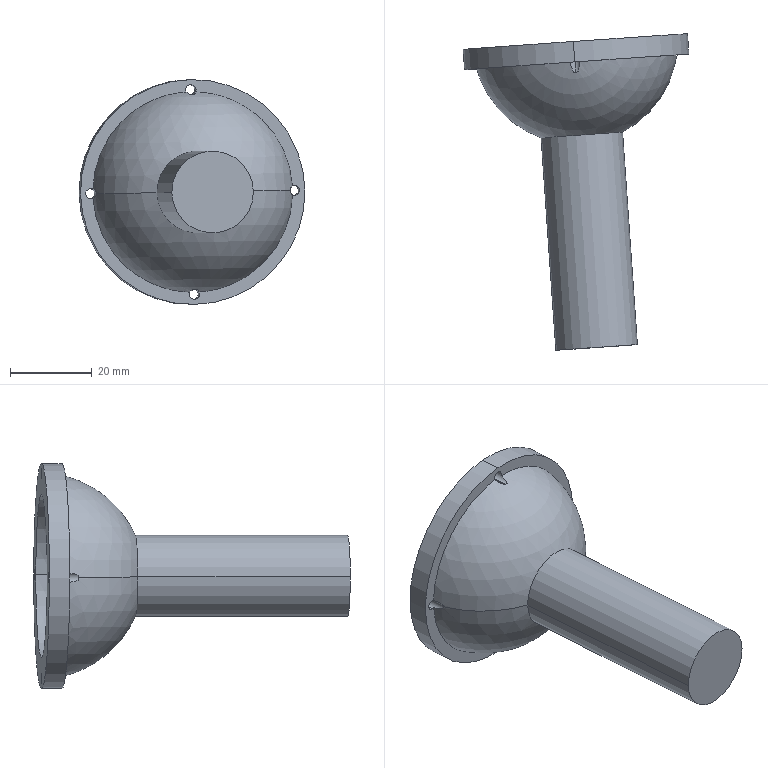Component | SolidWorks | ClampingMechanism-1_BallJointSeat-1 | 1 solid | 24 faces | box 55.21 x 77.43 x 55 mm | volume 34089 mm3 | cylinder 12 | cone 5 | sphere 4 | plane 3 | commonest cylinder face diameters 2.5 x8 55 x2 20 x2
STEP:
#1=COLOUR_RGB('',0.7922,0.8196,0.9333);
#2=FILL_AREA_STYLE_COLOUR('',#1);
#3=FILL_AREA_STYLE('',(#2));
#4=SURFACE_STYLE_FILL_AREA(#3);
#5=SURFACE_SIDE_STYLE('',(#4));
#6=SURFACE_STYLE_USAGE(.BOTH.,#5);
#7=PRESENTATION_STYLE_ASSIGNMENT((#6));
#8=CARTESIAN_POINT('',(2.771,-8.514,-22.315));
#9=VERTEX_POINT('',#8);
#10=CARTESIAN_POINT('',(2.789,-8.511,-22.315));
#11=VERTEX_POINT('',#10);
#12=CARTESIAN_POINT('',(2.771,-8.514,-22.315));
#13=CARTESIAN_POINT('',(2.777,-8.514,-22.315));
#14=CARTESIAN_POINT('',(2.783,-8.513,-22.315));
#15=CARTESIAN_POINT('',(2.789,-8.511,-22.315));
#16=B_SPLINE_CURVE_WITH_KNOTS('',3,(#12,#13,#14,#15),.UNSPECIFIED.,.F.,.F.,(4,4),(0.0004782,0.0009525),.UNSPECIFIED.);
#17=EDGE_CURVE('',#9,#11,#16,.T.);
#18=ORIENTED_EDGE('',*,*,#17,.F.);
#19=CARTESIAN_POINT('',(2.77,-8.512,-22.312));
#20=VERTEX_POINT('',#19);
#21=CARTESIAN_POINT('',(2.77,-8.512,-22.312));
#22=DIRECTION('',(-0.05098,0.5127,0.857));
#23=VECTOR('',#22,39.37);
#24=LINE('',#21,#23);
#25=EDGE_CURVE('',#9,#20,#24,.T.);
#26=ORIENTED_EDGE('',*,*,#25,.T.);
#27=CARTESIAN_POINT('',(2.771,-8.512,-22.361));
#28=DIRECTION('',(-0.06956,0.9976,0.));
#29=DIRECTION('',(-0.01767,-0.001232,0.9998));
#30=AXIS2_PLACEMENT_3D('',#27,#28,#29);
#31=CIRCLE('',#30,0.04921);
#32=EDGE_CURVE('',#20,#11,#31,.T.);
#33=ORIENTED_EDGE('',*,*,#32,.T.);
#34=EDGE_LOOP('',(#18,#26,#33));
#35=FACE_OUTER_BOUND('',#34,.T.);
#36=CARTESIAN_POINT('',(2.771,-8.512,-22.361));
#37=DIRECTION('',(-0.06956,0.9976,0.));
#38=DIRECTION('',(-0.01767,-0.001232,0.9998));
#39=AXIS2_PLACEMENT_3D('',#36,#37,#38);
#40=CONICAL_SURFACE('',#39,0.04921,1.03);
#41=ADVANCED_FACE('',(#35),#40,.F.);
#42=CARTESIAN_POINT('',(2.765,-8.414,-22.41));
#43=VERTEX_POINT('',#42);
#44=CARTESIAN_POINT('',(2.72,-8.417,-22.341));
#45=VERTEX_POINT('',#44);
#46=CARTESIAN_POINT('',(2.764,-8.414,-22.361));
#47=DIRECTION('',(-0.06956,0.9976,0.));
#48=DIRECTION('',(-0.01767,-0.001232,0.9998));
#49=AXIS2_PLACEMENT_3D('',#46,#47,#48);
#50=CIRCLE('',#49,0.04921);
#51=EDGE_CURVE('',#43,#45,#50,.T.);
#52=ORIENTED_EDGE('',*,*,#51,.F.);
#53=CARTESIAN_POINT('',(2.752,-8.218,-22.41));
#54=VERTEX_POINT('',#53);
#55=CARTESIAN_POINT('',(2.752,-8.218,-22.41));
#56=DIRECTION('',(-0.06956,0.9976,0.));
#57=VECTOR('',#56,39.37);
#58=LINE('',#55,#57);
#59=EDGE_CURVE('',#43,#54,#58,.T.);
#60=ORIENTED_EDGE('',*,*,#59,.T.);
#61=CARTESIAN_POINT('',(2.75,-8.218,-22.312));
#62=VERTEX_POINT('',#61);
#63=CARTESIAN_POINT('',(2.751,-8.218,-22.361));
#64=DIRECTION('',(-0.06956,0.9976,0.));
#65=DIRECTION('',(-0.01767,-0.001232,0.9998));
#66=AXIS2_PLACEMENT_3D('',#63,#64,#65);
#67=CIRCLE('',#66,0.04921);
#68=EDGE_CURVE('',#54,#62,#67,.T.);
#69=ORIENTED_EDGE('',*,*,#68,.T.);
#70=CARTESIAN_POINT('',(2.75,-8.218,-22.312));
#71=DIRECTION('',(-0.06956,0.9976,0.));
#72=VECTOR('',#71,39.37);
#73=LINE('',#70,#72);
#74=EDGE_CURVE('',#20,#62,#73,.T.);
#75=ORIENTED_EDGE('',*,*,#74,.F.);
#76=CARTESIAN_POINT('',(2.752,-8.514,-22.316));
#77=VERTEX_POINT('',#76);
#78=CARTESIAN_POINT('',(2.771,-8.512,-22.361));
#79=DIRECTION('',(-0.06956,0.9976,0.));
#80=DIRECTION('',(-0.01767,-0.001232,0.9998));
#81=AXIS2_PLACEMENT_3D('',#78,#79,#80);
#82=CIRCLE('',#81,0.04921);
#83=EDGE_CURVE('',#77,#20,#82,.T.);
#84=ORIENTED_EDGE('',*,*,#83,.F.);
#85=CARTESIAN_POINT('',(2.72,-8.417,-22.341));
#86=CARTESIAN_POINT('',(2.722,-8.434,-22.337));
#87=CARTESIAN_POINT('',(2.726,-8.451,-22.333));
#88=CARTESIAN_POINT('',(2.733,-8.476,-22.327));
#89=CARTESIAN_POINT('',(2.736,-8.484,-22.325));
#90=CARTESIAN_POINT('',(2.741,-8.495,-22.321));
#91=CARTESIAN_POINT('',(2.743,-8.499,-22.32));
#92=CARTESIAN_POINT('',(2.747,-8.507,-22.318));
#93=CARTESIAN_POINT('',(2.749,-8.51,-22.317));
#94=CARTESIAN_POINT('',(2.752,-8.514,-22.316));
#95=B_SPLINE_CURVE_WITH_KNOTS('',3,(#85,#86,#87,#88,#89,#90,#91,#92,#93,#94),.UNSPECIFIED.,.F.,.F.,(4,2,2,2,4),(0.0000002,0.00134,0.00201,0.002345,0.00268),.UNSPECIFIED.);
#96=EDGE_CURVE('',#45,#77,#95,.T.);
#97=ORIENTED_EDGE('',*,*,#96,.F.);
#98=EDGE_LOOP('',(#52,#60,#69,#75,#84,#97));
#99=FACE_OUTER_BOUND('',#98,.T.);
#100=CARTESIAN_POINT('',(2.751,-8.218,-22.361));
#101=DIRECTION('',(-0.06956,0.9976,0.));
#102=DIRECTION('',(-0.01767,-0.001232,0.9998));
#103=AXIS2_PLACEMENT_3D('',#100,#101,#102);
#104=CYLINDRICAL_SURFACE('',#103,0.04921);
#105=ADVANCED_FACE('',(#99),#104,.F.);
#106=CARTESIAN_POINT('',(3.73,-8.347,-21.409));
#107=VERTEX_POINT('',#106);
#108=CARTESIAN_POINT('',(3.709,-8.348,-21.404));
#109=VERTEX_POINT('',#108);
#110=CARTESIAN_POINT('',(3.729,-8.347,-21.359));
#111=DIRECTION('',(-0.06956,0.9976,0.));
#112=DIRECTION('',(-0.01767,-0.001232,0.9998));
#113=AXIS2_PLACEMENT_3D('',#110,#111,#112);
#114=CIRCLE('',#113,0.04921);
#115=EDGE_CURVE('',#107,#109,#114,.T.);
#116=ORIENTED_EDGE('',*,*,#115,.F.);
#117=CARTESIAN_POINT('',(3.716,-8.15,-21.409));
#118=VERTEX_POINT('',#117);
#119=CARTESIAN_POINT('',(3.716,-8.15,-21.409));
#120=DIRECTION('',(-0.06956,0.9976,0.));
#121=VECTOR('',#120,39.37);
#122=LINE('',#119,#121);
#123=EDGE_CURVE('',#107,#118,#122,.T.);
#124=ORIENTED_EDGE('',*,*,#123,.T.);
#125=CARTESIAN_POINT('',(3.714,-8.15,-21.31));
#126=VERTEX_POINT('',#125);
#127=CARTESIAN_POINT('',(3.715,-8.15,-21.359));
#128=DIRECTION('',(-0.06956,0.9976,0.));
#129=DIRECTION('',(-0.01767,-0.001232,0.9998));
#130=AXIS2_PLACEMENT_3D('',#127,#128,#129);
#131=CIRCLE('',#130,0.04921);
#132=EDGE_CURVE('',#118,#126,#131,.T.);
#133=ORIENTED_EDGE('',*,*,#132,.T.);
#134=CARTESIAN_POINT('',(3.728,-8.347,-21.31));
#135=VERTEX_POINT('',#134);
#136=CARTESIAN_POINT('',(3.714,-8.15,-21.31));
#137=DIRECTION('',(-0.06956,0.9976,0.));
#138=VECTOR('',#137,39.37);
#139=LINE('',#136,#138);
#140=EDGE_CURVE('',#135,#126,#139,.T.);
#141=ORIENTED_EDGE('',*,*,#140,.F.);
#142=CARTESIAN_POINT('',(3.707,-8.348,-21.315));
#143=VERTEX_POINT('',#142);
#144=CARTESIAN_POINT('',(3.729,-8.347,-21.359));
#145=DIRECTION('',(-0.06956,0.9976,0.));
#146=DIRECTION('',(-0.01767,-0.001232,0.9998));
#147=AXIS2_PLACEMENT_3D('',#144,#145,#146);
#148=CIRCLE('',#147,0.04921);
#149=EDGE_CURVE('',#143,#135,#148,.T.);
#150=ORIENTED_EDGE('',*,*,#149,.F.);
#151=CARTESIAN_POINT('',(3.69,-8.448,-21.341));
#152=VERTEX_POINT('',#151);
#153=CARTESIAN_POINT('',(3.69,-8.448,-21.341));
#154=CARTESIAN_POINT('',(3.691,-8.445,-21.339));
#155=CARTESIAN_POINT('',(3.691,-8.441,-21.337));
#156=CARTESIAN_POINT('',(3.693,-8.433,-21.333));
#157=CARTESIAN_POINT('',(3.694,-8.429,-21.331));
#158=CARTESIAN_POINT('',(3.696,-8.417,-21.327));
#159=CARTESIAN_POINT('',(3.698,-8.408,-21.325));
#160=CARTESIAN_POINT('',(3.702,-8.383,-21.319));
#161=CARTESIAN_POINT('',(3.705,-8.366,-21.317));
#162=CARTESIAN_POINT('',(3.707,-8.348,-21.315));
#163=B_SPLINE_CURVE_WITH_KNOTS('',3,(#153,#154,#155,#156,#157,#158,#159,#160,#161,#162),.UNSPECIFIED.,.F.,.F.,(4,2,2,2,4),(0.00000025,0.0003352,0.0006702,0.00134,0.00268),.UNSPECIFIED.);
#164=EDGE_CURVE('',#152,#143,#163,.T.);
#165=ORIENTED_EDGE('',*,*,#164,.F.);
#166=CARTESIAN_POINT('',(3.691,-8.448,-21.379));
#167=VERTEX_POINT('',#166);
#168=CARTESIAN_POINT('',(3.736,-8.445,-21.359));
#169=DIRECTION('',(-0.06956,0.9976,0.));
#170=DIRECTION('',(-0.01767,-0.001232,0.9998));
#171=AXIS2_PLACEMENT_3D('',#168,#169,#170);
#172=CIRCLE('',#171,0.04921);
#173=EDGE_CURVE('',#167,#152,#172,.T.);
#174=ORIENTED_EDGE('',*,*,#173,.F.);
#175=CARTESIAN_POINT('',(3.709,-8.348,-21.404));
#176=CARTESIAN_POINT('',(3.706,-8.366,-21.403));
#177=CARTESIAN_POINT('',(3.704,-8.383,-21.401));
#178=CARTESIAN_POINT('',(3.699,-8.408,-21.395));
#179=CARTESIAN_POINT('',(3.697,-8.417,-21.393));
#180=CARTESIAN_POINT('',(3.695,-8.429,-21.389));
#181=CARTESIAN_POINT('',(3.694,-8.433,-21.387));
#182=CARTESIAN_POINT('',(3.692,-8.441,-21.383));
#183=CARTESIAN_POINT('',(3.691,-8.444,-21.381));
#184=CARTESIAN_POINT('',(3.691,-8.448,-21.379));
#185=B_SPLINE_CURVE_WITH_KNOTS('',3,(#175,#176,#177,#178,#179,#180,#181,#182,#183,#184),.UNSPECIFIED.,.F.,.F.,(4,2,2,2,4),(0.0000002,0.00134,0.00201,0.002345,0.00268),.UNSPECIFIED.);
#186=EDGE_CURVE('',#109,#167,#185,.T.);
#187=ORIENTED_EDGE('',*,*,#186,.F.);
#188=EDGE_LOOP('',(#116,#124,#133,#141,#150,#165,#174,#187));
#189=FACE_OUTER_BOUND('',#188,.T.);
#190=CARTESIAN_POINT('',(3.715,-8.15,-21.359));
#191=DIRECTION('',(-0.06956,0.9976,0.));
#192=DIRECTION('',(-0.01767,-0.001232,0.9998));
#193=AXIS2_PLACEMENT_3D('',#190,#191,#192);
#194=CYLINDRICAL_SURFACE('',#193,0.04921);
#195=ADVANCED_FACE('',(#189),#194,.F.);
#196=CARTESIAN_POINT('',(2.737,-8.515,-20.442));
#197=VERTEX_POINT('',#196);
#198=CARTESIAN_POINT('',(2.719,-8.516,-20.439));
#199=VERTEX_POINT('',#198);
#200=CARTESIAN_POINT('',(2.736,-8.515,-20.393));
#201=DIRECTION('',(-0.06956,0.9976,0.));
#202=DIRECTION('',(-0.01767,-0.001232,0.9998));
#203=AXIS2_PLACEMENT_3D('',#200,#201,#202);
#204=CIRCLE('',#203,0.04921);
#205=EDGE_CURVE('',#197,#199,#204,.T.);
#206=ORIENTED_EDGE('',*,*,#205,.F.);
#207=CARTESIAN_POINT('',(2.717,-8.22,-20.442));
#208=VERTEX_POINT('',#207);
#209=CARTESIAN_POINT('',(2.717,-8.22,-20.442));
#210=DIRECTION('',(-0.06956,0.9976,0.));
#211=VECTOR('',#210,39.37);
#212=LINE('',#209,#211);
#213=EDGE_CURVE('',#197,#208,#212,.T.);
#214=ORIENTED_EDGE('',*,*,#213,.T.);
#215=CARTESIAN_POINT('',(2.715,-8.22,-20.343));
#216=VERTEX_POINT('',#215);
#217=CARTESIAN_POINT('',(2.716,-8.22,-20.393));
#218=DIRECTION('',(-0.06956,0.9976,0.));
#219=DIRECTION('',(-0.01767,-0.001232,0.9998));
#220=AXIS2_PLACEMENT_3D('',#217,#218,#219);
#221=CIRCLE('',#220,0.04921);
#222=EDGE_CURVE('',#208,#216,#221,.T.);
#223=ORIENTED_EDGE('',*,*,#222,.T.);
#224=CARTESIAN_POINT('',(2.729,-8.416,-20.343));
#225=VERTEX_POINT('',#224);
#226=CARTESIAN_POINT('',(2.715,-8.22,-20.343));
#227=DIRECTION('',(-0.06956,0.9976,0.));
#228=VECTOR('',#227,39.37);
#229=LINE('',#226,#228);
#230=EDGE_CURVE('',#225,#216,#229,.T.);
#231=ORIENTED_EDGE('',*,*,#230,.F.);
#232=CARTESIAN_POINT('',(2.686,-8.419,-20.414));
#233=VERTEX_POINT('',#232);
#234=CARTESIAN_POINT('',(2.73,-8.416,-20.393));
#235=DIRECTION('',(-0.06956,0.9976,0.));
#236=DIRECTION('',(-0.01767,-0.001232,0.9998));
#237=AXIS2_PLACEMENT_3D('',#234,#235,#236);
#238=CIRCLE('',#237,0.04921);
#239=EDGE_CURVE('',#233,#225,#238,.T.);
#240=ORIENTED_EDGE('',*,*,#239,.F.);
#241=CARTESIAN_POINT('',(2.719,-8.516,-20.439));
#242=CARTESIAN_POINT('',(2.716,-8.513,-20.438));
#243=CARTESIAN_POINT('',(2.713,-8.509,-20.436));
#244=CARTESIAN_POINT('',(2.709,-8.502,-20.434));
#245=CARTESIAN_POINT('',(2.707,-8.498,-20.433));
#246=CARTESIAN_POINT('',(2.702,-8.486,-20.43));
#247=CARTESIAN_POINT('',(2.699,-8.478,-20.428));
#248=CARTESIAN_POINT('',(2.692,-8.453,-20.422));
#249=CARTESIAN_POINT('',(2.688,-8.437,-20.418));
#250=CARTESIAN_POINT('',(2.686,-8.419,-20.414));
#251=B_SPLINE_CURVE_WITH_KNOTS('',3,(#241,#242,#243,#244,#245,#246,#247,#248,#249,#250),.UNSPECIFIED.,.F.,.F.,(4,2,2,2,4),(0.00000025,0.0003352,0.0006702,0.00134,0.00268),.UNSPECIFIED.);
#252=EDGE_CURVE('',#199,#233,#251,.T.);
#253=ORIENTED_EDGE('',*,*,#252,.F.);
#254=EDGE_LOOP('',(#206,#214,#223,#231,#240,#253));
#255=FACE_OUTER_BOUND('',#254,.T.);
#256=CARTESIAN_POINT('',(2.716,-8.22,-20.393));
#257=DIRECTION('',(-0.06956,0.9976,0.));
#258=DIRECTION('',(-0.01767,-0.001232,0.9998));
#259=AXIS2_PLACEMENT_3D('',#256,#257,#258);
#260=CYLINDRICAL_SURFACE('',#259,0.04921);
#261=ADVANCED_FACE('',(#255),#260,.F.);
#262=CARTESIAN_POINT('',(1.766,-8.484,-21.443));
#263=VERTEX_POINT('',#262);
#264=CARTESIAN_POINT('',(1.764,-8.484,-21.345));
#265=VERTEX_POINT('',#264);
#266=CARTESIAN_POINT('',(1.765,-8.484,-21.394));
#267=DIRECTION('',(-0.06956,0.9976,0.));
#268=DIRECTION('',(-0.01767,-0.001232,0.9998));
#269=AXIS2_PLACEMENT_3D('',#266,#267,#268);
#270=CIRCLE('',#269,0.04921);
#271=EDGE_CURVE('',#263,#265,#270,.T.);
#272=ORIENTED_EDGE('',*,*,#271,.F.);
#273=CARTESIAN_POINT('',(1.752,-8.287,-21.443));
#274=VERTEX_POINT('',#273);
#275=CARTESIAN_POINT('',(1.752,-8.287,-21.443));
#276=DIRECTION('',(-0.06956,0.9976,0.));
#277=VECTOR('',#276,39.37);
#278=LINE('',#275,#277);
#279=EDGE_CURVE('',#263,#274,#278,.T.);
#280=ORIENTED_EDGE('',*,*,#279,.T.);
#281=CARTESIAN_POINT('',(1.751,-8.287,-21.345));
#282=VERTEX_POINT('',#281);
#283=CARTESIAN_POINT('',(1.752,-8.287,-21.394));
#284=DIRECTION('',(-0.06956,0.9976,0.));
#285=DIRECTION('',(-0.01767,-0.001232,0.9998));
#286=AXIS2_PLACEMENT_3D('',#283,#284,#285);
#287=CIRCLE('',#286,0.04921);
#288=EDGE_CURVE('',#274,#282,#287,.T.);
#289=ORIENTED_EDGE('',*,*,#288,.T.);
#290=CARTESIAN_POINT('',(1.751,-8.287,-21.345));
#291=DIRECTION('',(-0.06956,0.9976,0.));
#292=VECTOR('',#291,39.37);
#293=LINE('',#290,#292);
#294=EDGE_CURVE('',#265,#282,#293,.T.);
#295=ORIENTED_EDGE('',*,*,#294,.F.);
#296=EDGE_LOOP('',(#272,#280,#289,#295));
#297=FACE_OUTER_BOUND('',#296,.T.);
#298=CARTESIAN_POINT('',(1.752,-8.287,-21.394));
#299=DIRECTION('',(-0.06956,0.9976,0.));
#300=DIRECTION('',(-0.01767,-0.001232,0.9998));
#301=AXIS2_PLACEMENT_3D('',#298,#299,#300);
#302=CYLINDRICAL_SURFACE('',#301,0.04921);
#303=ADVANCED_FACE('',(#297),#302,.F.);
#304=CARTESIAN_POINT('',(2.788,-9.004,-21.377));
#305=VERTEX_POINT('',#304);
#306=CARTESIAN_POINT('',(3.519,-8.164,-21.363));
#307=VERTEX_POINT('',#306);
#308=CARTESIAN_POINT('',(2.733,-8.219,-21.377));
#309=DIRECTION('',(-0.01767,-0.001232,0.9998));
#310=DIRECTION('',(0.9998,0.,0.01767));
#311=AXIS2_PLACEMENT_3D('',#308,#309,#310);
#312=CIRCLE('',#311,0.7874);
#313=EDGE_CURVE('',#305,#307,#312,.T.);
#314=ORIENTED_EDGE('',*,*,#313,.F.);
#315=CARTESIAN_POINT('',(1.948,-8.274,-21.391));
#316=VERTEX_POINT('',#315);
#317=CARTESIAN_POINT('',(2.733,-8.219,-21.377));
#318=DIRECTION('',(0.01767,0.001232,-0.9998));
#319=DIRECTION('',(-0.9998,0.,-0.01767));
#320=AXIS2_PLACEMENT_3D('',#317,#318,#319);
#321=CIRCLE('',#320,0.7874);
#322=EDGE_CURVE('',#305,#316,#321,.T.);
#323=ORIENTED_EDGE('',*,*,#322,.T.);
#324=CARTESIAN_POINT('',(2.733,-8.219,-21.377));
#325=DIRECTION('',(0.06956,-0.9976,-0.));
#326=DIRECTION('',(-0.01767,-0.001232,0.9998));
#327=AXIS2_PLACEMENT_3D('',#324,#325,#326);
#328=CIRCLE('',#327,0.7874);
#329=EDGE_CURVE('',#307,#316,#328,.T.);
#330=ORIENTED_EDGE('',*,*,#329,.F.);
#331=EDGE_LOOP('',(#314,#323,#330));
#332=FACE_OUTER_BOUND('',#331,.T.);
#333=CARTESIAN_POINT('',(2.733,-8.219,-21.377));
#334=DIRECTION('',(0.01767,0.001232,-0.9998));
#335=DIRECTION('',(0.9974,0.06955,0.01772));
#336=AXIS2_PLACEMENT_3D('',#333,#334,#335);
#337=SPHERICAL_SURFACE('',#336,0.7874);
#338=ADVANCED_FACE('',(#332),#337,.F.);
#339=CARTESIAN_POINT('',(2.728,-8.417,-20.294));
#340=VERTEX_POINT('',#339);
#341=CARTESIAN_POINT('',(2.766,-8.414,-22.459));
#342=VERTEX_POINT('',#341);
#343=CARTESIAN_POINT('',(2.747,-8.415,-21.377));
#344=DIRECTION('',(-0.06956,0.9976,0.));
#345=DIRECTION('',(-0.01767,-0.001232,0.9998));
#346=AXIS2_PLACEMENT_3D('',#343,#344,#345);
#347=CIRCLE('',#346,1.083);
#348=EDGE_CURVE('',#340,#342,#347,.T.);
#349=ORIENTED_EDGE('',*,*,#348,.T.);
#350=CARTESIAN_POINT('',(2.752,-8.217,-22.459));
#351=VERTEX_POINT('',#350);
#352=CARTESIAN_POINT('',(2.766,-8.414,-22.459));
#353=DIRECTION('',(-0.06956,0.9976,0.));
#354=VECTOR('',#353,39.37);
#355=LINE('',#352,#354);
#356=EDGE_CURVE('',#342,#351,#355,.T.);
#357=ORIENTED_EDGE('',*,*,#356,.T.);
#358=CARTESIAN_POINT('',(2.714,-8.22,-20.294));
#359=VERTEX_POINT('',#358);
#360=CARTESIAN_POINT('',(2.733,-8.219,-21.377));
#361=DIRECTION('',(-0.06956,0.9976,0.));
#362=DIRECTION('',(-0.01767,-0.001232,0.9998));
#363=AXIS2_PLACEMENT_3D('',#360,#361,#362);
#364=CIRCLE('',#363,1.083);
#365=EDGE_CURVE('',#359,#351,#364,.T.);
#366=ORIENTED_EDGE('',*,*,#365,.F.);
#367=CARTESIAN_POINT('',(2.728,-8.417,-20.294));
#368=DIRECTION('',(-0.06956,0.9976,0.));
#369=VECTOR('',#368,39.37);
#370=LINE('',#367,#369);
#371=EDGE_CURVE('',#340,#359,#370,.T.);
#372=ORIENTED_EDGE('',*,*,#371,.F.);
#373=EDGE_LOOP('',(#349,#357,#366,#372));
#374=FACE_OUTER_BOUND('',#373,.T.);
#375=CARTESIAN_POINT('',(2.747,-8.415,-21.377));
#376=DIRECTION('',(-0.06956,0.9976,0.));
#377=DIRECTION('',(-0.01767,-0.001232,0.9998));
#378=AXIS2_PLACEMENT_3D('',#375,#376,#377);
#379=CYLINDRICAL_SURFACE('',#378,1.083);
#380=ADVANCED_FACE('',(#374),#379,.T.);
#381=CARTESIAN_POINT('',(2.546,-11.192,-21.384));
#382=VERTEX_POINT('',#381);
#383=CARTESIAN_POINT('',(3.331,-11.137,-21.37));
#384=VERTEX_POINT('',#383);
#385=CARTESIAN_POINT('',(2.939,-11.164,-21.377));
#386=DIRECTION('',(-0.06956,0.9976,0.));
#387=DIRECTION('',(-0.9974,-0.06955,-0.01772));
#388=AXIS2_PLACEMENT_3D('',#385,#386,#387);
#389=CIRCLE('',#388,0.3937);
#390=EDGE_CURVE('',#382,#384,#389,.T.);
#391=ORIENTED_EDGE('',*,*,#390,.T.);
#392=CARTESIAN_POINT('',(3.189,-9.091,-21.37));
#393=VERTEX_POINT('',#392);
#394=CARTESIAN_POINT('',(3.058,-7.21,-21.37));
#395=DIRECTION('',(-0.06956,0.9976,0.));
#396=VECTOR('',#395,39.37);
#397=LINE('',#394,#396);
#398=EDGE_CURVE('',#384,#393,#397,.T.);
#399=ORIENTED_EDGE('',*,*,#398,.T.);
#400=CARTESIAN_POINT('',(2.403,-9.146,-21.384));
#401=VERTEX_POINT('',#400);
#402=CARTESIAN_POINT('',(2.796,-9.119,-21.377));
#403=DIRECTION('',(-0.06956,0.9976,0.));
#404=DIRECTION('',(-0.9974,-0.06955,-0.01772));
#405=AXIS2_PLACEMENT_3D('',#402,#403,#404);
#406=CIRCLE('',#405,0.3937);
#407=EDGE_CURVE('',#401,#393,#406,.T.);
#408=ORIENTED_EDGE('',*,*,#407,.F.);
#409=CARTESIAN_POINT('',(2.272,-7.264,-21.384));
#410=DIRECTION('',(-0.06956,0.9976,0.));
#411=VECTOR('',#410,39.37);
#412=LINE('',#409,#411);
#413=EDGE_CURVE('',#382,#401,#412,.T.);
#414=ORIENTED_EDGE('',*,*,#413,.F.);
#415=EDGE_LOOP('',(#391,#399,#408,#414));
#416=FACE_OUTER_BOUND('',#415,.T.);
#417=CARTESIAN_POINT('',(2.665,-7.237,-21.377));
#418=DIRECTION('',(-0.06956,0.9976,0.));
#419=DIRECTION('',(-0.9974,-0.06955,-0.01772));
#420=AXIS2_PLACEMENT_3D('',#417,#418,#419);
#421=CYLINDRICAL_SURFACE('',#420,0.3937);
#422=ADVANCED_FACE('',(#416),#421,.T.);
#423=CARTESIAN_POINT('',(2.796,-9.119,-21.377));
#424=DIRECTION('',(-0.06956,0.9976,0.));
#425=DIRECTION('',(-0.9974,-0.06955,-0.01772));
#426=AXIS2_PLACEMENT_3D('',#423,#424,#425);
#427=CIRCLE('',#426,0.3937);
#428=EDGE_CURVE('',#393,#401,#427,.T.);
#429=ORIENTED_EDGE('',*,*,#428,.T.);
#430=CARTESIAN_POINT('',(1.818,-8.581,-21.393));
#431=VERTEX_POINT('',#430);
#432=CARTESIAN_POINT('',(2.733,-8.219,-21.377));
#433=DIRECTION('',(0.01767,0.001232,-0.9998));
#434=DIRECTION('',(-0.9998,0.,-0.01767));
#435=AXIS2_PLACEMENT_3D('',#432,#433,#434);
#436=CIRCLE('',#435,0.9843);
#437=EDGE_CURVE('',#401,#431,#436,.T.);
#438=ORIENTED_EDGE('',*,*,#437,.T.);
#439=CARTESIAN_POINT('',(1.818,-8.579,-21.412));
#440=VERTEX_POINT('',#439);
#441=CARTESIAN_POINT('',(1.818,-8.581,-21.393));
#442=CARTESIAN_POINT('',(1.818,-8.581,-21.4));
#443=CARTESIAN_POINT('',(1.818,-8.58,-21.406));
#444=CARTESIAN_POINT('',(1.818,-8.579,-21.412));
#445=B_SPLINE_CURVE_WITH_KNOTS('',3,(#441,#442,#443,#444),.UNSPECIFIED.,.F.,.F.,(4,4),(0.0004782,0.0009525),.UNSPECIFIED.);
#446=EDGE_CURVE('',#431,#440,#445,.T.);
#447=ORIENTED_EDGE('',*,*,#446,.T.);
#448=CARTESIAN_POINT('',(1.787,-8.482,-21.438));
#449=VERTEX_POINT('',#448);
#450=CARTESIAN_POINT('',(1.818,-8.579,-21.412));
#451=CARTESIAN_POINT('',(1.817,-8.575,-21.415));
#452=CARTESIAN_POINT('',(1.815,-8.572,-21.417));
#453=CARTESIAN_POINT('',(1.813,-8.564,-21.421));
#454=CARTESIAN_POINT('',(1.811,-8.56,-21.422));
#455=CARTESIAN_POINT('',(1.807,-8.548,-21.427));
#456=CARTESIAN_POINT('',(1.804,-8.54,-21.429));
#457=CARTESIAN_POINT('',(1.797,-8.516,-21.434));
#458=CARTESIAN_POINT('',(1.792,-8.499,-21.437));
#459=CARTESIAN_POINT('',(1.787,-8.482,-21.438));
#460=B_SPLINE_CURVE_WITH_KNOTS('',3,(#450,#451,#452,#453,#454,#455,#456,#457,#458,#459),.UNSPECIFIED.,.F.,.F.,(4,2,2,2,4),(0.00000025,0.0003352,0.0006702,0.00134,0.00268),.UNSPECIFIED.);
#461=EDGE_CURVE('',#440,#449,#460,.T.);
#462=ORIENTED_EDGE('',*,*,#461,.T.);
#463=CARTESIAN_POINT('',(2.747,-8.415,-21.377));
#464=DIRECTION('',(-0.06956,0.9976,0.));
#465=DIRECTION('',(-0.01767,-0.001232,0.9998));
#466=AXIS2_PLACEMENT_3D('',#463,#464,#465);
#467=CIRCLE('',#466,0.9644);
#468=EDGE_CURVE('',#45,#449,#467,.T.);
#469=ORIENTED_EDGE('',*,*,#468,.F.);
#470=ORIENTED_EDGE('',*,*,#96,.T.);
#471=CARTESIAN_POINT('',(2.752,-8.514,-22.316));
#472=CARTESIAN_POINT('',(2.758,-8.514,-22.315));
#473=CARTESIAN_POINT('',(2.764,-8.515,-22.315));
#474=CARTESIAN_POINT('',(2.771,-8.514,-22.315));
#475=B_SPLINE_CURVE_WITH_KNOTS('',3,(#471,#472,#473,#474),.UNSPECIFIED.,.F.,.F.,(4,4),(0.00000099,0.0004782),.UNSPECIFIED.);
#476=EDGE_CURVE('',#77,#9,#475,.T.);
#477=ORIENTED_EDGE('',*,*,#476,.T.);
#478=ORIENTED_EDGE('',*,*,#17,.T.);
#479=CARTESIAN_POINT('',(2.808,-8.411,-22.339));
#480=VERTEX_POINT('',#479);
#481=CARTESIAN_POINT('',(2.789,-8.511,-22.315));
#482=CARTESIAN_POINT('',(2.791,-8.507,-22.316));
#483=CARTESIAN_POINT('',(2.793,-8.503,-22.317));
#484=CARTESIAN_POINT('',(2.796,-8.495,-22.319));
#485=CARTESIAN_POINT('',(2.798,-8.491,-22.32));
#486=CARTESIAN_POINT('',(2.801,-8.479,-22.324));
#487=CARTESIAN_POINT('',(2.803,-8.471,-22.326));
#488=CARTESIAN_POINT('',(2.807,-8.445,-22.332));
#489=CARTESIAN_POINT('',(2.808,-8.428,-22.336));
#490=CARTESIAN_POINT('',(2.808,-8.411,-22.339));
#491=B_SPLINE_CURVE_WITH_KNOTS('',3,(#481,#482,#483,#484,#485,#486,#487,#488,#489,#490),.UNSPECIFIED.,.F.,.F.,(4,2,2,2,4),(0.00000025,0.0003352,0.0006702,0.00134,0.00268),.UNSPECIFIED.);
#492=EDGE_CURVE('',#11,#480,#491,.T.);
#493=ORIENTED_EDGE('',*,*,#492,.T.);
#494=CARTESIAN_POINT('',(2.747,-8.415,-21.377));
#495=DIRECTION('',(-0.06956,0.9976,0.));
#496=DIRECTION('',(-0.01767,-0.001232,0.9998));
#497=AXIS2_PLACEMENT_3D('',#494,#495,#496);
#498=CIRCLE('',#497,0.9644);
#499=EDGE_CURVE('',#109,#480,#498,.T.);
#500=ORIENTED_EDGE('',*,*,#499,.F.);
#501=ORIENTED_EDGE('',*,*,#186,.T.);
#502=CARTESIAN_POINT('',(3.69,-8.45,-21.36));
#503=VERTEX_POINT('',#502);
#504=CARTESIAN_POINT('',(3.691,-8.448,-21.379));
#505=CARTESIAN_POINT('',(3.69,-8.449,-21.373));
#506=CARTESIAN_POINT('',(3.69,-8.45,-21.366));
#507=CARTESIAN_POINT('',(3.69,-8.45,-21.36));
#508=B_SPLINE_CURVE_WITH_KNOTS('',3,(#504,#505,#506,#507),.UNSPECIFIED.,.F.,.F.,(4,4),(0.00000099,0.0004782),.UNSPECIFIED.);
#509=EDGE_CURVE('',#167,#503,#508,.T.);
#510=ORIENTED_EDGE('',*,*,#509,.T.);
#511=CARTESIAN_POINT('',(2.733,-8.219,-21.377));
#512=DIRECTION('',(-0.01767,-0.001232,0.9998));
#513=DIRECTION('',(0.9998,0.,0.01767));
#514=AXIS2_PLACEMENT_3D('',#511,#512,#513);
#515=CIRCLE('',#514,0.9843);
#516=EDGE_CURVE('',#393,#503,#515,.T.);
#517=ORIENTED_EDGE('',*,*,#516,.F.);
#518=EDGE_LOOP('',(#429,#438,#447,#462,#469,#470,#477,#478,#493,#500,#501,#510,#517));
#519=FACE_OUTER_BOUND('',#518,.T.);
#520=CARTESIAN_POINT('',(2.733,-8.219,-21.377));
#521=DIRECTION('',(0.01767,0.001232,-0.9998));
#522=DIRECTION('',(0.9974,0.06955,0.01772));
#523=AXIS2_PLACEMENT_3D('',#520,#521,#522);
#524=SPHERICAL_SURFACE('',#523,0.9843);
#525=ADVANCED_FACE('',(#519),#524,.T.);
#526=ORIENTED_EDGE('',*,*,#437,.F.);
#527=ORIENTED_EDGE('',*,*,#407,.T.);
#528=ORIENTED_EDGE('',*,*,#516,.T.);
#529=CARTESIAN_POINT('',(3.69,-8.45,-21.36));
#530=CARTESIAN_POINT('',(3.69,-8.45,-21.354));
#531=CARTESIAN_POINT('',(3.69,-8.449,-21.348));
#532=CARTESIAN_POINT('',(3.69,-8.448,-21.341));
#533=B_SPLINE_CURVE_WITH_KNOTS('',3,(#529,#530,#531,#532),.UNSPECIFIED.,.F.,.F.,(4,4),(0.0004782,0.0009525),.UNSPECIFIED.);
#534=EDGE_CURVE('',#503,#152,#533,.T.);
#535=ORIENTED_EDGE('',*,*,#534,.T.);
#536=ORIENTED_EDGE('',*,*,#164,.T.);
#537=CARTESIAN_POINT('',(2.774,-8.413,-20.413));
#538=VERTEX_POINT('',#537);
#539=CARTESIAN_POINT('',(2.747,-8.415,-21.377));
#540=DIRECTION('',(-0.06956,0.9976,0.));
#541=DIRECTION('',(-0.01767,-0.001232,0.9998));
#542=AXIS2_PLACEMENT_3D('',#539,#540,#541);
#543=CIRCLE('',#542,0.9644);
#544=EDGE_CURVE('',#538,#143,#543,.T.);
#545=ORIENTED_EDGE('',*,*,#544,.F.);
#546=CARTESIAN_POINT('',(2.756,-8.513,-20.438));
#547=VERTEX_POINT('',#546);
#548=CARTESIAN_POINT('',(2.774,-8.413,-20.413));
#549=CARTESIAN_POINT('',(2.774,-8.431,-20.416));
#550=CARTESIAN_POINT('',(2.773,-8.448,-20.42));
#551=CARTESIAN_POINT('',(2.769,-8.473,-20.427));
#552=CARTESIAN_POINT('',(2.768,-8.482,-20.429));
#553=CARTESIAN_POINT('',(2.764,-8.494,-20.432));
#554=CARTESIAN_POINT('',(2.763,-8.498,-20.433));
#555=CARTESIAN_POINT('',(2.76,-8.506,-20.436));
#556=CARTESIAN_POINT('',(2.758,-8.51,-20.437));
#557=CARTESIAN_POINT('',(2.756,-8.513,-20.438));
#558=B_SPLINE_CURVE_WITH_KNOTS('',3,(#548,#549,#550,#551,#552,#553,#554,#555,#556,#557),.UNSPECIFIED.,.F.,.F.,(4,2,2,2,4),(0.0000002,0.00134,0.00201,0.002345,0.00268),.UNSPECIFIED.);
#559=EDGE_CURVE('',#538,#547,#558,.T.);
#560=ORIENTED_EDGE('',*,*,#559,.T.);
#561=CARTESIAN_POINT('',(2.756,-8.513,-20.438));
#562=CARTESIAN_POINT('',(2.75,-8.515,-20.438));
#563=CARTESIAN_POINT('',(2.744,-8.516,-20.439));
#564=CARTESIAN_POINT('',(2.731,-8.517,-20.439));
#565=CARTESIAN_POINT('',(2.725,-8.517,-20.439));
#566=CARTESIAN_POINT('',(2.719,-8.516,-20.439));
#567=B_SPLINE_CURVE_WITH_KNOTS('',3,(#561,#562,#563,#564,#565,#566),.UNSPECIFIED.,.F.,.F.,(4,2,4),(0.00000099,0.0004767,0.0009525),.UNSPECIFIED.);
#568=EDGE_CURVE('',#547,#199,#567,.T.);
#569=ORIENTED_EDGE('',*,*,#568,.T.);
#570=ORIENTED_EDGE('',*,*,#252,.T.);
#571=CARTESIAN_POINT('',(1.785,-8.482,-21.349));
#572=VERTEX_POINT('',#571);
#573=CARTESIAN_POINT('',(2.747,-8.415,-21.377));
#574=DIRECTION('',(-0.06956,0.9976,0.));
#575=DIRECTION('',(-0.01767,-0.001232,0.9998));
#576=AXIS2_PLACEMENT_3D('',#573,#574,#575);
#577=CIRCLE('',#576,0.9644);
#578=EDGE_CURVE('',#572,#233,#577,.T.);
#579=ORIENTED_EDGE('',*,*,#578,.F.);
#580=CARTESIAN_POINT('',(1.817,-8.579,-21.375));
#581=VERTEX_POINT('',#580);
#582=CARTESIAN_POINT('',(1.785,-8.482,-21.349));
#583=CARTESIAN_POINT('',(1.79,-8.499,-21.351));
#584=CARTESIAN_POINT('',(1.795,-8.516,-21.353));
#585=CARTESIAN_POINT('',(1.803,-8.54,-21.358));
#586=CARTESIAN_POINT('',(1.806,-8.549,-21.361));
#587=CARTESIAN_POINT('',(1.81,-8.56,-21.365));
#588=CARTESIAN_POINT('',(1.812,-8.564,-21.366));
#589=CARTESIAN_POINT('',(1.815,-8.572,-21.37));
#590=CARTESIAN_POINT('',(1.816,-8.575,-21.372));
#591=CARTESIAN_POINT('',(1.817,-8.579,-21.375));
#592=B_SPLINE_CURVE_WITH_KNOTS('',3,(#582,#583,#584,#585,#586,#587,#588,#589,#590,#591),.UNSPECIFIED.,.F.,.F.,(4,2,2,2,4),(0.0000002,0.00134,0.00201,0.002345,0.00268),.UNSPECIFIED.);
#593=EDGE_CURVE('',#572,#581,#592,.T.);
#594=ORIENTED_EDGE('',*,*,#593,.T.);
#595=CARTESIAN_POINT('',(1.817,-8.579,-21.375));
#596=CARTESIAN_POINT('',(1.818,-8.58,-21.381));
#597=CARTESIAN_POINT('',(1.818,-8.581,-21.387));
#598=CARTESIAN_POINT('',(1.818,-8.581,-21.393));
#599=B_SPLINE_CURVE_WITH_KNOTS('',3,(#595,#596,#597,#598),.UNSPECIFIED.,.F.,.F.,(4,4),(0.00000099,0.0004782),.UNSPECIFIED.);
#600=EDGE_CURVE('',#581,#431,#599,.T.);
#601=ORIENTED_EDGE('',*,*,#600,.T.);
#602=EDGE_LOOP('',(#526,#527,#528,#535,#536,#545,#560,#569,#570,#579,#594,#601));
#603=FACE_OUTER_BOUND('',#602,.T.);
#604=CARTESIAN_POINT('',(2.733,-8.219,-21.377));
#605=DIRECTION('',(0.01767,0.001232,-0.9998));
#606=DIRECTION('',(0.9974,0.06955,0.01772));
#607=AXIS2_PLACEMENT_3D('',#604,#605,#606);
#608=SPHERICAL_SURFACE('',#607,0.9843);
#609=ADVANCED_FACE('',(#603),#608,.T.);
#610=ORIENTED_EDGE('',*,*,#390,.F.);
#611=CARTESIAN_POINT('',(2.939,-11.164,-21.377));
#612=DIRECTION('',(-0.06956,0.9976,0.));
#613=DIRECTION('',(-0.9974,-0.06955,-0.01772));
#614=AXIS2_PLACEMENT_3D('',#611,#612,#613);
#615=CIRCLE('',#614,0.3937);
#616=EDGE_CURVE('',#384,#382,#615,.T.);
#617=ORIENTED_EDGE('',*,*,#616,.F.);
#618=EDGE_LOOP('',(#610,#617));
#619=FACE_OUTER_BOUND('',#618,.T.);
#620=CARTESIAN_POINT('',(2.939,-11.164,-21.377));
#621=DIRECTION('',(-0.06956,0.9976,0.));
#622=DIRECTION('',(-0.9974,-0.06955,-0.01772));
#623=AXIS2_PLACEMENT_3D('',#620,#621,#622);
#624=PLANE('',#623);
#625=ADVANCED_FACE('',(#619),#624,.F.);
#626=ORIENTED_EDGE('',*,*,#398,.F.);
#627=ORIENTED_EDGE('',*,*,#616,.T.);
#628=ORIENTED_EDGE('',*,*,#413,.T.);
#629=ORIENTED_EDGE('',*,*,#428,.F.);
#630=EDGE_LOOP('',(#626,#627,#628,#629));
#631=FACE_OUTER_BOUND('',#630,.T.);
#632=CARTESIAN_POINT('',(2.665,-7.237,-21.377));
#633=DIRECTION('',(-0.06956,0.9976,0.));
#634=DIRECTION('',(-0.9974,-0.06955,-0.01772));
#635=AXIS2_PLACEMENT_3D('',#632,#633,#634);
#636=CYLINDRICAL_SURFACE('',#635,0.3937);
#637=ADVANCED_FACE('',(#631),#636,.T.);
#638=ORIENTED_EDGE('',*,*,#356,.F.);
#639=CARTESIAN_POINT('',(2.747,-8.415,-21.377));
#640=DIRECTION('',(-0.06956,0.9976,0.));
#641=DIRECTION('',(-0.01767,-0.001232,0.9998));
#642=AXIS2_PLACEMENT_3D('',#639,#640,#641);
#643=CIRCLE('',#642,1.083);
#644=EDGE_CURVE('',#342,#340,#643,.T.);
#645=ORIENTED_EDGE('',*,*,#644,.T.);
#646=ORIENTED_EDGE('',*,*,#371,.T.);
#647=CARTESIAN_POINT('',(2.733,-8.219,-21.377));
#648=DIRECTION('',(-0.06956,0.9976,0.));
#649=DIRECTION('',(-0.01767,-0.001232,0.9998));
#650=AXIS2_PLACEMENT_3D('',#647,#648,#649);
#651=CIRCLE('',#650,1.083);
#652=EDGE_CURVE('',#351,#359,#651,.T.);
#653=ORIENTED_EDGE('',*,*,#652,.F.);
#654=EDGE_LOOP('',(#638,#645,#646,#653));
#655=FACE_OUTER_BOUND('',#654,.T.);
#656=CARTESIAN_POINT('',(2.747,-8.415,-21.377));
#657=DIRECTION('',(-0.06956,0.9976,0.));
#658=DIRECTION('',(-0.01767,-0.001232,0.9998));
#659=AXIS2_PLACEMENT_3D('',#656,#657,#658);
#660=CYLINDRICAL_SURFACE('',#659,1.083);
#661=ADVANCED_FACE('',(#655),#660,.T.);
#662=ORIENTED_EDGE('',*,*,#499,.T.);
#663=CARTESIAN_POINT('',(2.764,-8.414,-22.361));
#664=DIRECTION('',(-0.06956,0.9976,0.));
#665=DIRECTION('',(-0.01767,-0.001232,0.9998));
#666=AXIS2_PLACEMENT_3D('',#663,#664,#665);
#667=CIRCLE('',#666,0.04921);
#668=EDGE_CURVE('',#480,#43,#667,.T.);
#669=ORIENTED_EDGE('',*,*,#668,.T.);
#670=ORIENTED_EDGE('',*,*,#51,.T.);
#671=ORIENTED_EDGE('',*,*,#468,.T.);
#672=CARTESIAN_POINT('',(1.765,-8.484,-21.394));
#673=DIRECTION('',(-0.06956,0.9976,0.));
#674=DIRECTION('',(-0.01767,-0.001232,0.9998));
#675=AXIS2_PLACEMENT_3D('',#672,#673,#674);
#676=CIRCLE('',#675,0.04921);
#677=EDGE_CURVE('',#449,#263,#676,.T.);
#678=ORIENTED_EDGE('',*,*,#677,.T.);
#679=ORIENTED_EDGE('',*,*,#271,.T.);
#680=CARTESIAN_POINT('',(1.765,-8.484,-21.394));
#681=DIRECTION('',(-0.06956,0.9976,0.));
#682=DIRECTION('',(-0.01767,-0.001232,0.9998));
#683=AXIS2_PLACEMENT_3D('',#680,#681,#682);
#684=CIRCLE('',#683,0.04921);
#685=EDGE_CURVE('',#265,#572,#684,.T.);
#686=ORIENTED_EDGE('',*,*,#685,.T.);
#687=ORIENTED_EDGE('',*,*,#578,.T.);
#688=ORIENTED_EDGE('',*,*,#239,.T.);
#689=CARTESIAN_POINT('',(2.73,-8.416,-20.393));
#690=DIRECTION('',(-0.06956,0.9976,0.));
#691=DIRECTION('',(-0.01767,-0.001232,0.9998));
#692=AXIS2_PLACEMENT_3D('',#689,#690,#691);
#693=CIRCLE('',#692,0.04921);
#694=EDGE_CURVE('',#225,#538,#693,.T.);
#695=ORIENTED_EDGE('',*,*,#694,.T.);
#696=ORIENTED_EDGE('',*,*,#544,.T.);
#697=ORIENTED_EDGE('',*,*,#149,.T.);
#698=CARTESIAN_POINT('',(3.729,-8.347,-21.359));
#699=DIRECTION('',(-0.06956,0.9976,0.));
#700=DIRECTION('',(-0.01767,-0.001232,0.9998));
#701=AXIS2_PLACEMENT_3D('',#698,#699,#700);
#702=CIRCLE('',#701,0.04921);
#703=EDGE_CURVE('',#135,#107,#702,.T.);
#704=ORIENTED_EDGE('',*,*,#703,.T.);
#705=ORIENTED_EDGE('',*,*,#115,.T.);
#706=EDGE_LOOP('',(#662,#669,#670,#671,#678,#679,#686,#687,#688,#695,#696,#697,#704,#705));
#707=FACE_BOUND('',#706,.T.);
#708=ORIENTED_EDGE('',*,*,#348,.F.);
#709=ORIENTED_EDGE('',*,*,#644,.F.);
#710=EDGE_LOOP('',(#708,#709));
#711=FACE_OUTER_BOUND('',#710,.T.);
#712=CARTESIAN_POINT('',(2.747,-8.415,-21.377));
#713=DIRECTION('',(-0.06956,0.9976,0.));
#714=DIRECTION('',(-0.01767,-0.001232,0.9998));
#715=AXIS2_PLACEMENT_3D('',#712,#713,#714);
#716=PLANE('',#715);
#717=ADVANCED_FACE('',(#707,#711),#716,.F.);
#718=ORIENTED_EDGE('',*,*,#322,.F.);
#719=ORIENTED_EDGE('',*,*,#313,.T.);
#720=CARTESIAN_POINT('',(2.733,-8.219,-21.377));
#721=DIRECTION('',(0.06956,-0.9976,-0.));
#722=DIRECTION('',(-0.01767,-0.001232,0.9998));
#723=AXIS2_PLACEMENT_3D('',#720,#721,#722);
#724=CIRCLE('',#723,0.7874);
#725=EDGE_CURVE('',#316,#307,#724,.T.);
#726=ORIENTED_EDGE('',*,*,#725,.F.);
#727=EDGE_LOOP('',(#718,#719,#726));
#728=FACE_OUTER_BOUND('',#727,.T.);
#729=CARTESIAN_POINT('',(2.733,-8.219,-21.377));
#730=DIRECTION('',(0.01767,0.001232,-0.9998));
#731=DIRECTION('',(0.9974,0.06955,0.01772));
#732=AXIS2_PLACEMENT_3D('',#729,#730,#731);
#733=SPHERICAL_SURFACE('',#732,0.7874);
#734=ADVANCED_FACE('',(#728),#733,.F.);
#735=CARTESIAN_POINT('',(2.751,-8.218,-22.361));
#736=DIRECTION('',(-0.06956,0.9976,0.));
#737=DIRECTION('',(-0.01767,-0.001232,0.9998));
#738=AXIS2_PLACEMENT_3D('',#735,#736,#737);
#739=CIRCLE('',#738,0.04921);
#740=EDGE_CURVE('',#62,#54,#739,.T.);
#741=ORIENTED_EDGE('',*,*,#740,.F.);
#742=ORIENTED_EDGE('',*,*,#68,.F.);
#743=EDGE_LOOP('',(#741,#742));
#744=FACE_BOUND('',#743,.T.);
#745=CARTESIAN_POINT('',(3.715,-8.15,-21.359));
#746=DIRECTION('',(-0.06956,0.9976,0.));
#747=DIRECTION('',(-0.01767,-0.001232,0.9998));
#748=AXIS2_PLACEMENT_3D('',#745,#746,#747);
#749=CIRCLE('',#748,0.04921);
#750=EDGE_CURVE('',#126,#118,#749,.T.);
#751=ORIENTED_EDGE('',*,*,#750,.F.);
#752=ORIENTED_EDGE('',*,*,#132,.F.);
#753=EDGE_LOOP('',(#751,#752));
#754=FACE_BOUND('',#753,.T.);
#755=CARTESIAN_POINT('',(2.716,-8.22,-20.393));
#756=DIRECTION('',(-0.06956,0.9976,0.));
#757=DIRECTION('',(-0.01767,-0.001232,0.9998));
#758=AXIS2_PLACEMENT_3D('',#755,#756,#757);
#759=CIRCLE('',#758,0.04921);
#760=EDGE_CURVE('',#216,#208,#759,.T.);
#761=ORIENTED_EDGE('',*,*,#760,.F.);
#762=ORIENTED_EDGE('',*,*,#222,.F.);
#763=EDGE_LOOP('',(#761,#762));
#764=FACE_BOUND('',#763,.T.);
#765=CARTESIAN_POINT('',(1.752,-8.287,-21.394));
#766=DIRECTION('',(-0.06956,0.9976,0.));
#767=DIRECTION('',(-0.01767,-0.001232,0.9998));
#768=AXIS2_PLACEMENT_3D('',#765,#766,#767);
#769=CIRCLE('',#768,0.04921);
#770=EDGE_CURVE('',#282,#274,#769,.T.);
#771=ORIENTED_EDGE('',*,*,#770,.F.);
#772=ORIENTED_EDGE('',*,*,#288,.F.);
#773=EDGE_LOOP('',(#771,#772));
#774=FACE_BOUND('',#773,.T.);
#775=ORIENTED_EDGE('',*,*,#329,.T.);
#776=ORIENTED_EDGE('',*,*,#725,.T.);
#777=EDGE_LOOP('',(#775,#776));
#778=FACE_BOUND('',#777,.T.);
#779=ORIENTED_EDGE('',*,*,#365,.T.);
#780=ORIENTED_EDGE('',*,*,#652,.T.);
#781=EDGE_LOOP('',(#779,#780));
#782=FACE_OUTER_BOUND('',#781,.T.);
#783=CARTESIAN_POINT('',(2.733,-8.219,-21.377));
#784=DIRECTION('',(-0.06956,0.9976,0.));
#785=DIRECTION('',(-0.01767,-0.001232,0.9998));
#786=AXIS2_PLACEMENT_3D('',#783,#784,#785);
#787=PLANE('',#786);
#788=ADVANCED_FACE('',(#744,#754,#764,#774,#778,#782),#787,.T.);
#789=ORIENTED_EDGE('',*,*,#279,.F.);
#790=ORIENTED_EDGE('',*,*,#677,.F.);
#791=ORIENTED_EDGE('',*,*,#461,.F.);
#792=CARTESIAN_POINT('',(1.772,-8.582,-21.394));
#793=DIRECTION('',(-0.06956,0.9976,0.));
#794=DIRECTION('',(-0.01767,-0.001232,0.9998));
#795=AXIS2_PLACEMENT_3D('',#792,#793,#794);
#796=CIRCLE('',#795,0.04921);
#797=EDGE_CURVE('',#581,#440,#796,.T.);
#798=ORIENTED_EDGE('',*,*,#797,.F.);
#799=ORIENTED_EDGE('',*,*,#593,.F.);
#800=ORIENTED_EDGE('',*,*,#685,.F.);
#801=ORIENTED_EDGE('',*,*,#294,.T.);
#802=ORIENTED_EDGE('',*,*,#770,.T.);
#803=EDGE_LOOP('',(#789,#790,#791,#798,#799,#800,#801,#802));
#804=FACE_OUTER_BOUND('',#803,.T.);
#805=CARTESIAN_POINT('',(1.752,-8.287,-21.394));
#806=DIRECTION('',(-0.06956,0.9976,0.));
#807=DIRECTION('',(-0.01767,-0.001232,0.9998));
#808=AXIS2_PLACEMENT_3D('',#805,#806,#807);
#809=CYLINDRICAL_SURFACE('',#808,0.04921);
#810=ADVANCED_FACE('',(#804),#809,.F.);
#811=ORIENTED_EDGE('',*,*,#797,.T.);
#812=ORIENTED_EDGE('',*,*,#446,.F.);
#813=ORIENTED_EDGE('',*,*,#600,.F.);
#814=EDGE_LOOP('',(#811,#812,#813));
#815=FACE_OUTER_BOUND('',#814,.T.);
#816=CARTESIAN_POINT('',(1.772,-8.582,-21.394));
#817=DIRECTION('',(-0.06956,0.9976,0.));
#818=DIRECTION('',(-0.01767,-0.001232,0.9998));
#819=AXIS2_PLACEMENT_3D('',#816,#817,#818);
#820=CONICAL_SURFACE('',#819,0.04921,1.03);
#821=ADVANCED_FACE('',(#815),#820,.F.);
#822=ORIENTED_EDGE('',*,*,#213,.F.);
#823=CARTESIAN_POINT('',(2.736,-8.515,-20.393));
#824=DIRECTION('',(-0.06956,0.9976,0.));
#825=DIRECTION('',(-0.01767,-0.001232,0.9998));
#826=AXIS2_PLACEMENT_3D('',#823,#824,#825);
#827=CIRCLE('',#826,0.04921);
#828=EDGE_CURVE('',#547,#197,#827,.T.);
#829=ORIENTED_EDGE('',*,*,#828,.F.);
#830=ORIENTED_EDGE('',*,*,#559,.F.);
#831=ORIENTED_EDGE('',*,*,#694,.F.);
#832=ORIENTED_EDGE('',*,*,#230,.T.);
#833=ORIENTED_EDGE('',*,*,#760,.T.);
#834=EDGE_LOOP('',(#822,#829,#830,#831,#832,#833));
#835=FACE_OUTER_BOUND('',#834,.T.);
#836=CARTESIAN_POINT('',(2.716,-8.22,-20.393));
#837=DIRECTION('',(-0.06956,0.9976,0.));
#838=DIRECTION('',(-0.01767,-0.001232,0.9998));
#839=AXIS2_PLACEMENT_3D('',#836,#837,#838);
#840=CYLINDRICAL_SURFACE('',#839,0.04921);
#841=ADVANCED_FACE('',(#835),#840,.F.);
#842=ORIENTED_EDGE('',*,*,#828,.T.);
#843=ORIENTED_EDGE('',*,*,#205,.T.);
#844=ORIENTED_EDGE('',*,*,#568,.F.);
#845=EDGE_LOOP('',(#842,#843,#844));
#846=FACE_OUTER_BOUND('',#845,.T.);
#847=CARTESIAN_POINT('',(2.736,-8.515,-20.393));
#848=DIRECTION('',(-0.06956,0.9976,0.));
#849=DIRECTION('',(-0.01767,-0.001232,0.9998));
#850=AXIS2_PLACEMENT_3D('',#847,#848,#849);
#851=CONICAL_SURFACE('',#850,0.04921,1.03);
#852=ADVANCED_FACE('',(#846),#851,.F.);
#853=ORIENTED_EDGE('',*,*,#123,.F.);
#854=ORIENTED_EDGE('',*,*,#703,.F.);
#855=ORIENTED_EDGE('',*,*,#140,.T.);
#856=ORIENTED_EDGE('',*,*,#750,.T.);
#857=EDGE_LOOP('',(#853,#854,#855,#856));
#858=FACE_OUTER_BOUND('',#857,.T.);
#859=CARTESIAN_POINT('',(3.715,-8.15,-21.359));
#860=DIRECTION('',(-0.06956,0.9976,0.));
#861=DIRECTION('',(-0.01767,-0.001232,0.9998));
#862=AXIS2_PLACEMENT_3D('',#859,#860,#861);
#863=CYLINDRICAL_SURFACE('',#862,0.04921);
#864=ADVANCED_FACE('',(#858),#863,.F.);
#865=ORIENTED_EDGE('',*,*,#173,.T.);
#866=ORIENTED_EDGE('',*,*,#534,.F.);
#867=ORIENTED_EDGE('',*,*,#509,.F.);
#868=EDGE_LOOP('',(#865,#866,#867));
#869=FACE_OUTER_BOUND('',#868,.T.);
#870=CARTESIAN_POINT('',(3.736,-8.445,-21.359));
#871=DIRECTION('',(-0.06956,0.9976,0.));
#872=DIRECTION('',(-0.01767,-0.001232,0.9998));
#873=AXIS2_PLACEMENT_3D('',#870,#871,#872);
#874=CONICAL_SURFACE('',#873,0.04921,1.03);
#875=ADVANCED_FACE('',(#869),#874,.F.);
#876=ORIENTED_EDGE('',*,*,#59,.F.);
#877=ORIENTED_EDGE('',*,*,#668,.F.);
#878=ORIENTED_EDGE('',*,*,#492,.F.);
#879=ORIENTED_EDGE('',*,*,#32,.F.);
#880=ORIENTED_EDGE('',*,*,#74,.T.);
#881=ORIENTED_EDGE('',*,*,#740,.T.);
#882=EDGE_LOOP('',(#876,#877,#878,#879,#880,#881));
#883=FACE_OUTER_BOUND('',#882,.T.);
#884=CARTESIAN_POINT('',(2.751,-8.218,-22.361));
#885=DIRECTION('',(-0.06956,0.9976,0.));
#886=DIRECTION('',(-0.01767,-0.001232,0.9998));
#887=AXIS2_PLACEMENT_3D('',#884,#885,#886);
#888=CYLINDRICAL_SURFACE('',#887,0.04921);
#889=ADVANCED_FACE('',(#883),#888,.F.);
#890=ORIENTED_EDGE('',*,*,#25,.F.);
#891=ORIENTED_EDGE('',*,*,#476,.F.);
#892=ORIENTED_EDGE('',*,*,#83,.T.);
#893=EDGE_LOOP('',(#890,#891,#892));
#894=FACE_OUTER_BOUND('',#893,.T.);
#895=CARTESIAN_POINT('',(2.771,-8.512,-22.361));
#896=DIRECTION('',(-0.06956,0.9976,0.));
#897=DIRECTION('',(-0.01767,-0.001232,0.9998));
#898=AXIS2_PLACEMENT_3D('',#895,#896,#897);
#899=CONICAL_SURFACE('',#898,0.04921,1.03);
#900=ADVANCED_FACE('',(#894),#899,.F.);
#901=CLOSED_SHELL('',(#41,#105,#195,#261,#303,#338,#380,#422,#525,#609,#625,#637,#661,#717,#734,#788,#810,#821,#841,#852,#864,#875,#889,#900));
#902=MANIFOLD_SOLID_BREP('',#901);
#903=STYLED_ITEM('',(#7),#902);
#904=PRESENTATION_LAYER_ASSIGNMENT('','',(#903));
#905=(LENGTH_UNIT()NAMED_UNIT(*)SI_UNIT($,.METRE.));
#906=LENGTH_MEASURE_WITH_UNIT(LENGTH_MEASURE(0.0254),#905);
#907=DIMENSIONAL_EXPONENTS(1.,0.,0.,0.,0.,0.,0.);
#908=(CONVERSION_BASED_UNIT('',#906)LENGTH_UNIT()NAMED_UNIT(#907));
#909=UNCERTAINTY_MEASURE_WITH_UNIT(LENGTH_MEASURE(0.00001),#908,'','');
#910=(NAMED_UNIT(*)PLANE_ANGLE_UNIT()SI_UNIT($,.RADIAN.));
#911=(NAMED_UNIT(*)SI_UNIT($,.STERADIAN.)SOLID_ANGLE_UNIT());
#912=(GEOMETRIC_REPRESENTATION_CONTEXT(3)GLOBAL_UNCERTAINTY_ASSIGNED_CONTEXT((#909))GLOBAL_UNIT_ASSIGNED_CONTEXT((#908,#910,#911))REPRESENTATION_CONTEXT('',''));
#913=MECHANICAL_DESIGN_GEOMETRIC_PRESENTATION_REPRESENTATION('',(#903),#912);
#914=CARTESIAN_POINT('',(0.,0.,0.));
#915=DIRECTION('',(0.,0.,1.));
#916=DIRECTION('',(1.,0.,0.));
#917=AXIS2_PLACEMENT_3D('',#914,#915,#916);
#918=(LENGTH_UNIT()NAMED_UNIT(*)SI_UNIT($,.METRE.));
#919=LENGTH_MEASURE_WITH_UNIT(LENGTH_MEASURE(0.0254),#918);
#920=DIMENSIONAL_EXPONENTS(1.,0.,0.,0.,0.,0.,0.);
#921=(CONVERSION_BASED_UNIT('',#919)LENGTH_UNIT()NAMED_UNIT(#920));
#922=UNCERTAINTY_MEASURE_WITH_UNIT(LENGTH_MEASURE(0.00001),#921,'','');
#923=(NAMED_UNIT(*)PLANE_ANGLE_UNIT()SI_UNIT($,.RADIAN.));
#924=(NAMED_UNIT(*)SI_UNIT($,.STERADIAN.)SOLID_ANGLE_UNIT());
#925=(GEOMETRIC_REPRESENTATION_CONTEXT(3)GLOBAL_UNCERTAINTY_ASSIGNED_CONTEXT((#922))GLOBAL_UNIT_ASSIGNED_CONTEXT((#921,#923,#924))REPRESENTATION_CONTEXT('',''));
#926=ADVANCED_BREP_SHAPE_REPRESENTATION('',(#902,#917),#925);